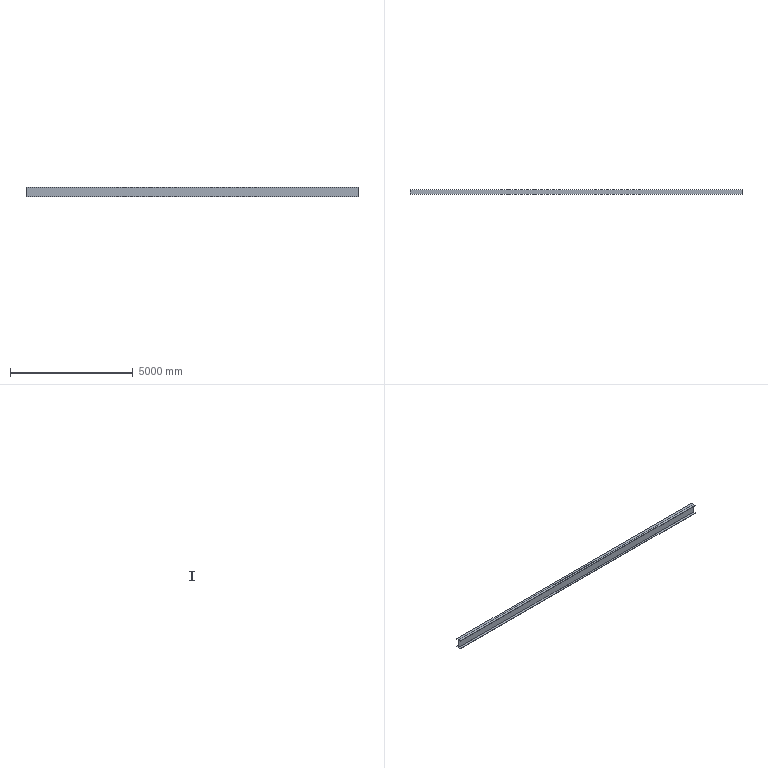Component | NX | 6_10 | 1 solid | 14 faces | volume 110592000 mm3 | plane 14